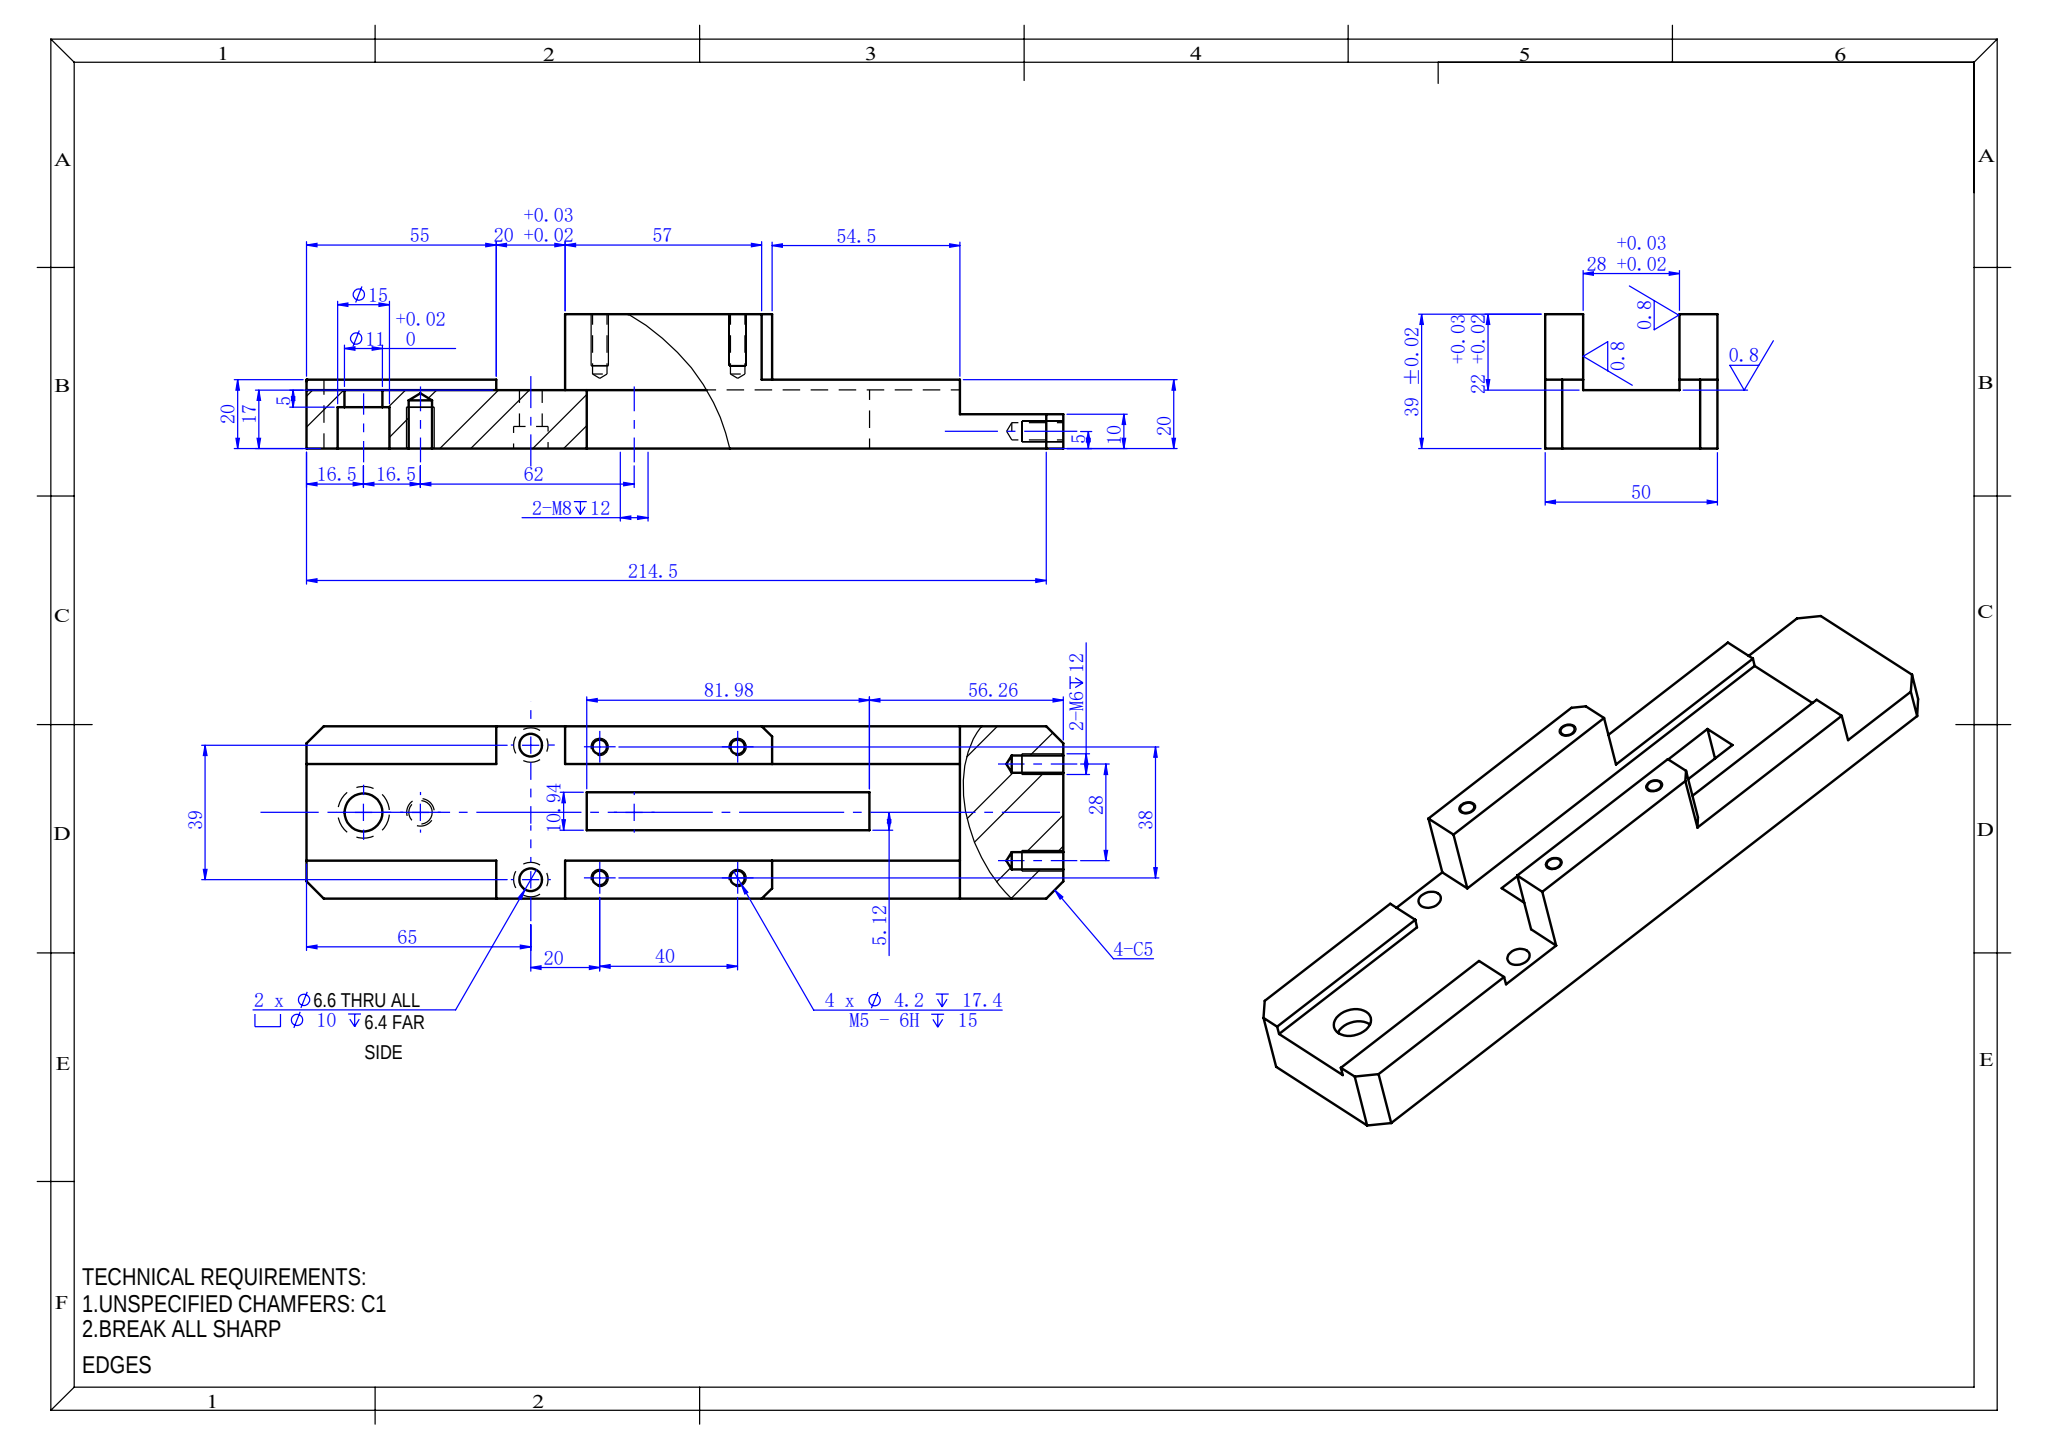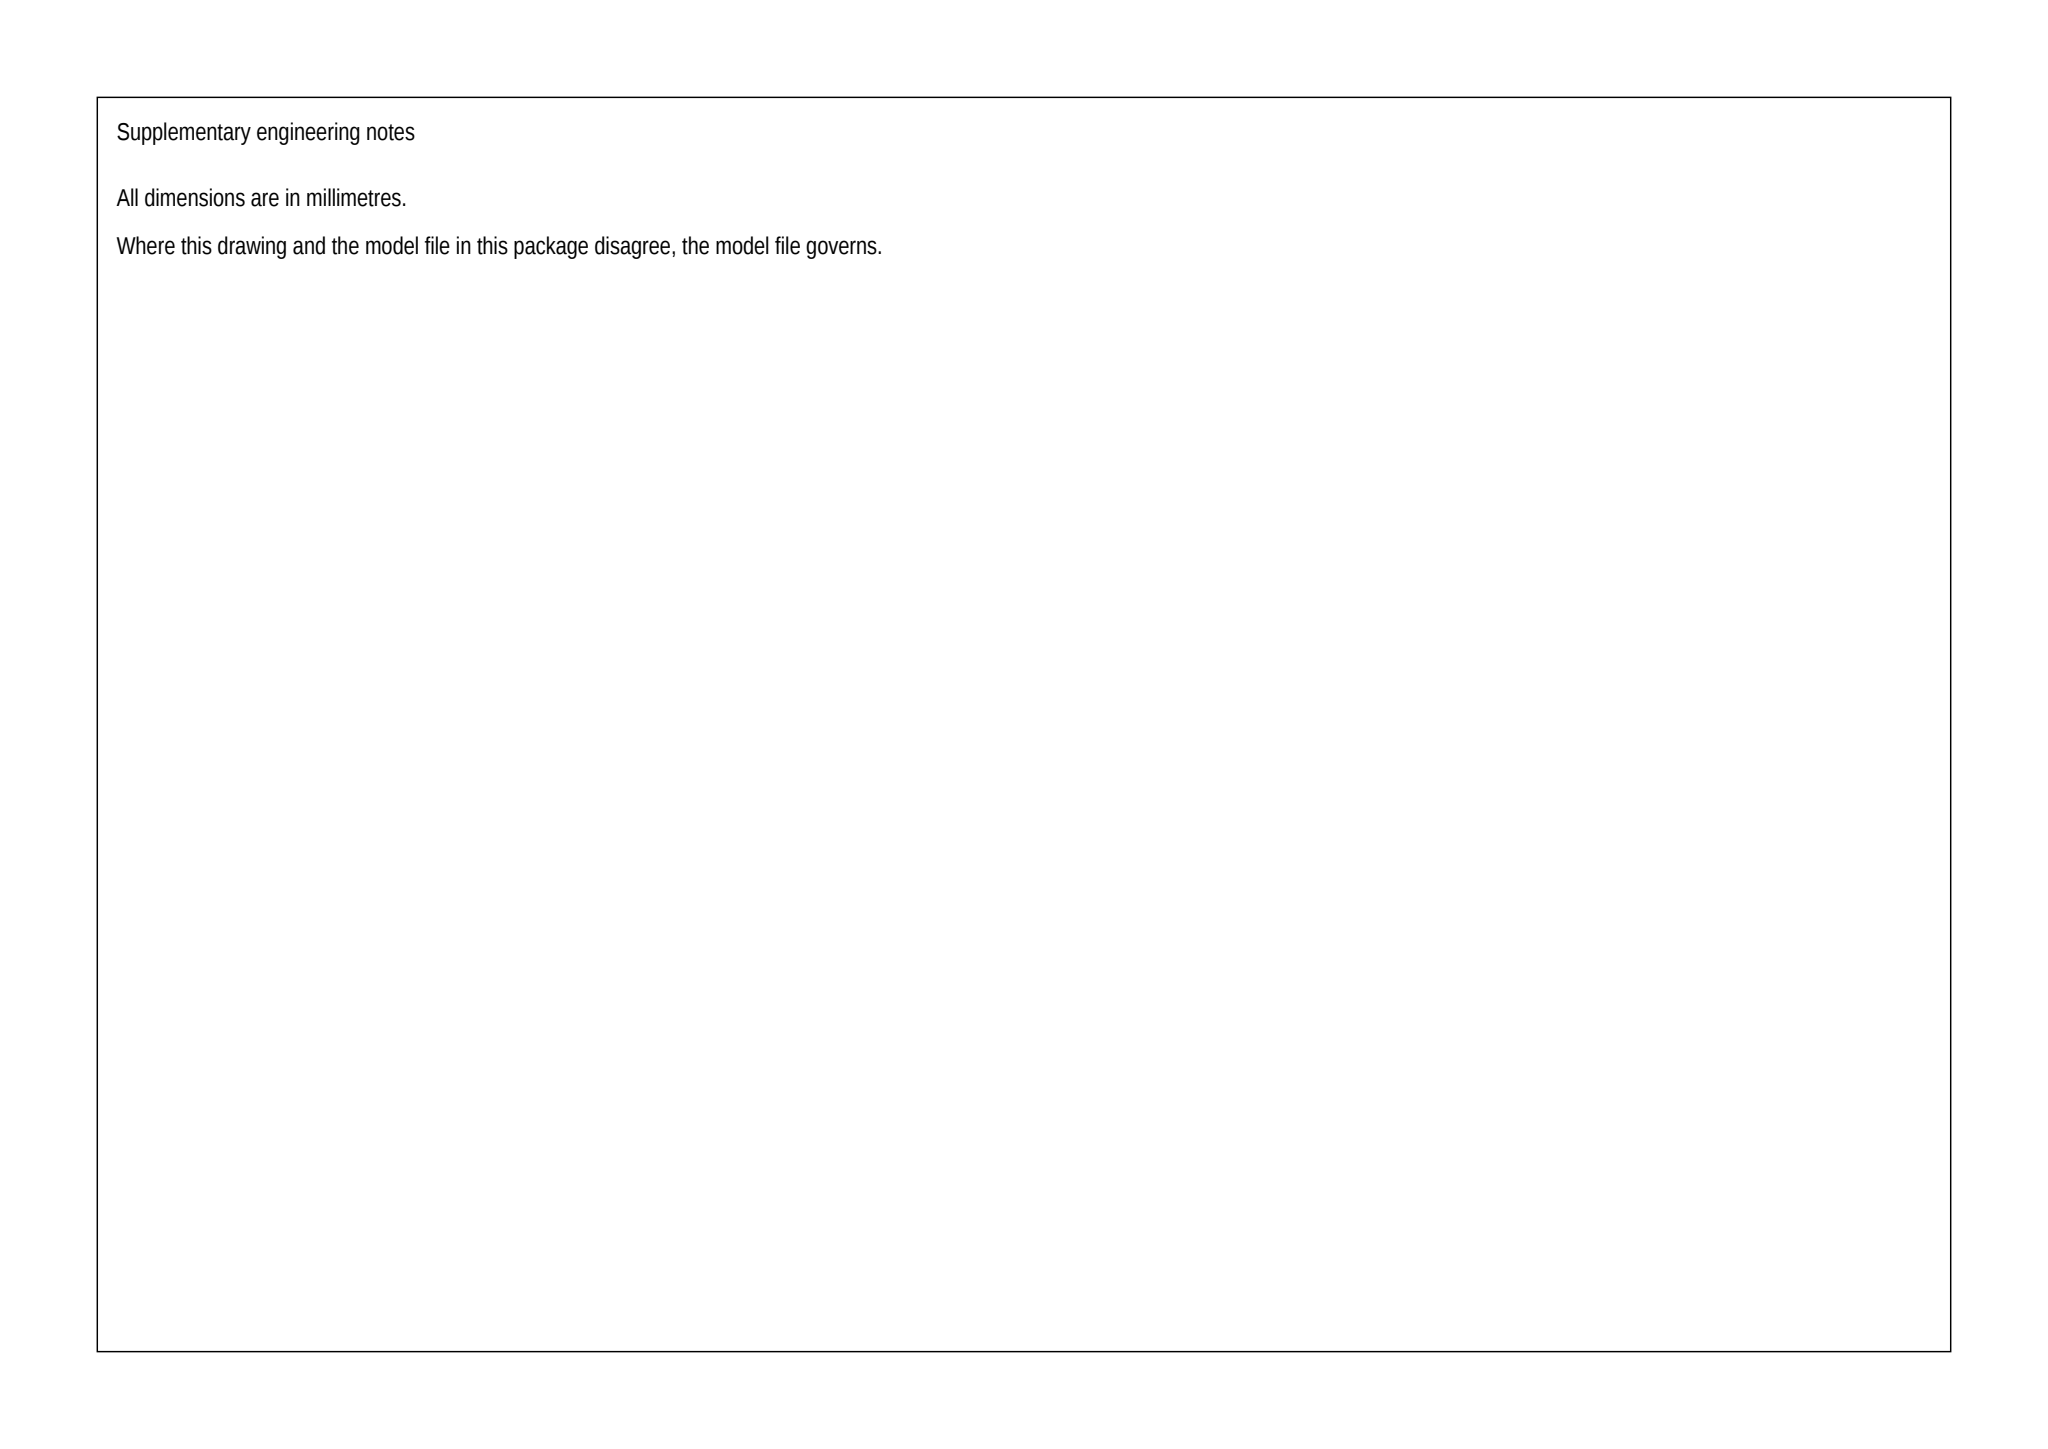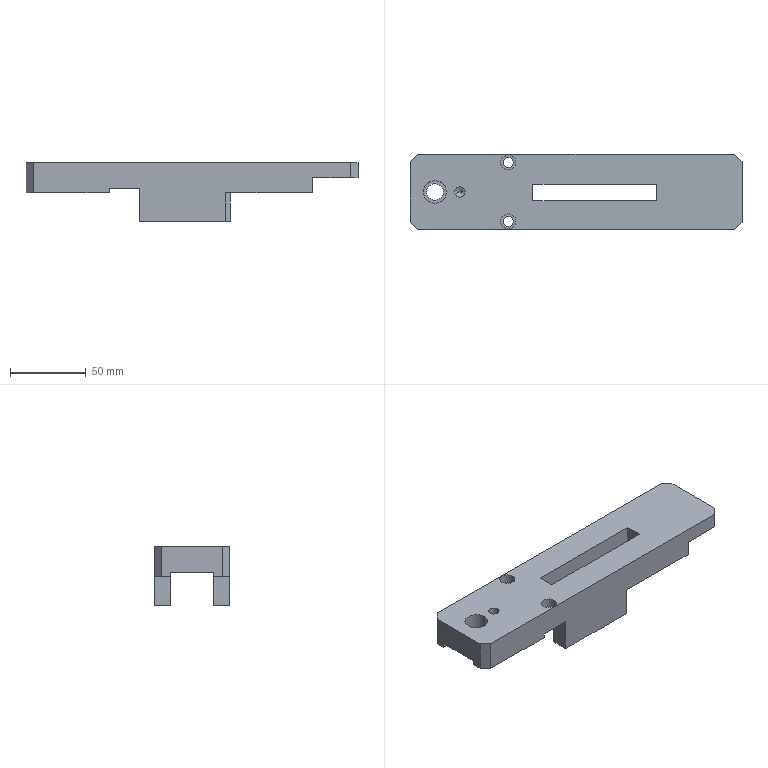Part | SolidWorks | mm | 1 solid | 77 faces | box 219.5 x 50 x 39 mm | volume 189716 mm3 | plane 37 | cylinder 26 | cone 14 | commonest cylinder face diameters 4.2 x8 10 x4 6.6 x4 5 x4 6.8 x2 15 x2 11 x2
build123d program:
from build123d import *

# Parameters (mm, degrees)
SKETCH1_W                                       = 219.5
SKETCH1_H                                       = 50
BOSS_EXTRUDE1_DEPTH                             = 20
SKETCH2_W                                       = 20
SKETCH2_H                                       = 3
CUT_EXTRUDE1_DEPTH                              = 125.756
SKETCH3_W                                       = 3
SKETCH3_H                                       = 28
CUT_EXTRUDE2_DEPTH                              = 227.452
SKETCH6_R                                       = 5.5
CUT_EXTRUDE5_DEPTH                              = 126.113
SKETCH7_R                                       = 7.5
CUT_EXTRUDE6_DEPTH                              = 12
SKETCH8_W                                       = 60
SKETCH8_H                                       = 11
BOSS_EXTRUDE2_DEPTH                             = 19
SKETCH9_W                                       = 30
SKETCH9_H                                       = 10
CUT_EXTRUDE7_DEPTH                              = 125.756
CHAMFER1_SIZE                                   = 3
M6_TAPPED_HOLE3_D                               = 5
M6_TAPPED_HOLE3_DEPTH                           = 15
M6_TAPPED_HOLE3_TIP                             = 1.502
M6_HEX_SOCKET_HEAD_CAP_SCREW_CBORE4_D           = 6.6
M6_HEX_SOCKET_HEAD_CAP_SCREW_CBORE4_CBORE_D     = 10
M6_HEX_SOCKET_HEAD_CAP_SCREW_CBORE4_CBORE_DEPTH = 6.4
M8_TAPPED_HOLE1_D                               = 6.8
M8_TAPPED_HOLE1_DEPTH                           = 14
M8_TAPPED_HOLE1_TIP                             = 2.043
M5_TAPPED_HOLE1_D                               = 4.2
M5_TAPPED_HOLE1_DEPTH                           = 17.4
M5_TAPPED_HOLE1_TIP                             = 1.262
CHAMFER2_SIZE                                   = 5
SKETCH27_W                                      = 81.979
SKETCH27_H                                      = 10.942
CUT_EXTRUDE8_DEPTH                              = 36


with BuildPart() as part:
    # Sketch1 → Boss-Extrude1 (new body)
    with BuildSketch(Plane.XY):
        with Locations((-2.785, 26.964)):
            Rectangle(SKETCH1_W, SKETCH1_H)
    extrude(amount=BOSS_EXTRUDE1_DEPTH)

    # Sketch2 → Cut-Extrude1 (cut, through all)
    with BuildSketch(Plane(origin=(0, 1.964, 0), x_dir=(-1, 0, 0), z_dir=(0, -1, 0))):
        with Locations((47.535, -1.5)):
            Rectangle(SKETCH2_W, SKETCH2_H)
    extrude(amount=-CUT_EXTRUDE1_DEPTH, mode=Mode.SUBTRACT)

    # Sketch3 → Cut-Extrude2 (cut, through all)
    with BuildSketch(Plane.ZY.offset(112.535)):
        with Locations((1.5, 26.964)):
            Rectangle(SKETCH3_W, SKETCH3_H)
    extrude(amount=-CUT_EXTRUDE2_DEPTH, mode=Mode.SUBTRACT)

    # Sketch6 → Cut-Extrude5 (cut, through all)
    with BuildSketch(Plane(origin=(0, 0, 3), x_dir=(-1, 0, 0), z_dir=(0, 0, -1))):
        with Locations((96.035, 26.964)):
            Circle(SKETCH6_R)
    extrude(amount=-CUT_EXTRUDE5_DEPTH, mode=Mode.SUBTRACT)

    # Sketch7 → Cut-Extrude6 (cut)
    with BuildSketch(Plane.XY.offset(20)):
        with Locations((-96.035, 26.964)):
            Circle(SKETCH7_R)
    extrude(amount=-CUT_EXTRUDE6_DEPTH, mode=Mode.SUBTRACT)

    # Sketch8 → Boss-Extrude2 (add)
    with BuildSketch(Plane(origin=(0, 0, 0), x_dir=(-1, 0, 0), z_dir=(0, 0, -1))):
        with Locations((7.535, 46.464)):
            Rectangle(SKETCH8_W, SKETCH8_H)
        with Locations((7.535, 7.464)):
            Rectangle(SKETCH8_W, SKETCH8_H)
    extrude(amount=BOSS_EXTRUDE2_DEPTH)

    # Sketch9 → Cut-Extrude7 (cut, through all)
    with BuildSketch(Plane(origin=(0, 51.964, 0), x_dir=(1, 0, 0), z_dir=(0, 1, 0))):
        with Locations((91.965, -5)):
            Rectangle(SKETCH9_W, SKETCH9_H)
    extrude(amount=-CUT_EXTRUDE7_DEPTH, mode=Mode.SUBTRACT)

    # Chamfer1
    chamfer1_edges = [part.edges().sort_by_distance(p)[0] for p in [
        (22.465, 51.964, -9.5),
        (22.465, 1.964, -9.5),
    ]]
    chamfer(chamfer1_edges, length=CHAMFER1_SIZE)

    # M6 Tapped Hole3
    with Locations(Plane(origin=(106.965, 0, 0), x_dir=(0, 0, -1), z_dir=(1, 0, 0))):
        with Locations((-15, 40.964), (-15, 12.964)):
            Hole(M6_TAPPED_HOLE3_D / 2, depth=M6_TAPPED_HOLE3_DEPTH)
            with Locations((0, 0, -(M6_TAPPED_HOLE3_DEPTH + M6_TAPPED_HOLE3_TIP / 2))):  # 118° drill point
                Cone(0, M6_TAPPED_HOLE3_D / 2, M6_TAPPED_HOLE3_TIP, mode=Mode.SUBTRACT)

    # M6 Hex Socket Head Cap Screw CBORE4 (through all)
    with Locations(Plane.XY.offset(20)):
        with Locations((-47.535, 7.464), (-47.535, 46.464)):
            CounterBoreHole(M6_HEX_SOCKET_HEAD_CAP_SCREW_CBORE4_D / 2, M6_HEX_SOCKET_HEAD_CAP_SCREW_CBORE4_CBORE_D / 2, M6_HEX_SOCKET_HEAD_CAP_SCREW_CBORE4_CBORE_DEPTH)

    # M8 Tapped Hole1
    with Locations(Plane.XY.offset(20)):
        with Locations((-17.535, 26.964), (-79.535, 26.964)):
            Hole(M8_TAPPED_HOLE1_D / 2, depth=M8_TAPPED_HOLE1_DEPTH)
            with Locations((0, 0, -(M8_TAPPED_HOLE1_DEPTH + M8_TAPPED_HOLE1_TIP / 2))):  # 118° drill point
                Cone(0, M8_TAPPED_HOLE1_D / 2, M8_TAPPED_HOLE1_TIP, mode=Mode.SUBTRACT)

    # M5 Tapped Hole1
    with Locations(Plane(origin=(0, 0, -19), x_dir=(-1, 0, 0), z_dir=(0, 0, -1))):
        with Locations((27.535, 7.964), (-12.465, 7.964), (-12.465, 45.964), (27.535, 45.964)):
            Hole(M5_TAPPED_HOLE1_D / 2, depth=M5_TAPPED_HOLE1_DEPTH)
            with Locations((0, 0, -(M5_TAPPED_HOLE1_DEPTH + M5_TAPPED_HOLE1_TIP / 2))):  # 118° drill point
                Cone(0, M5_TAPPED_HOLE1_D / 2, M5_TAPPED_HOLE1_TIP, mode=Mode.SUBTRACT)

    # Chamfer2
    chamfer2_edges = [part.edges().sort_by_distance(p)[0] for p in [
        (-112.535, 51.964, 10),
        (106.965, 51.964, 15),
        (106.965, 1.964, 15),
        (-112.535, 1.964, 10),
    ]]
    chamfer(chamfer2_edges, length=CHAMFER2_SIZE)

    # Sketch27 → Cut-Extrude8 (cut)
    with BuildSketch(Plane(origin=(0, 0, 3), x_dir=(-1, 0, 0), z_dir=(0, 0, -1))):
        with Locations((-9.721, 26.616)):
            Rectangle(SKETCH27_W, SKETCH27_H)
    extrude(amount=-CUT_EXTRUDE8_DEPTH, mode=Mode.SUBTRACT)


solid = part.part